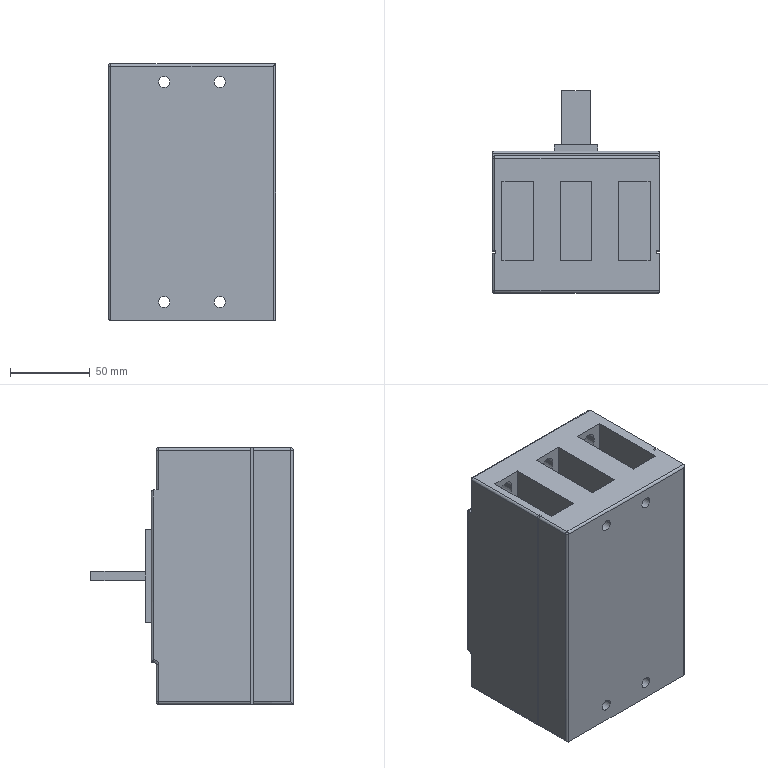Component | SolidWorks | NSX100F-3PMoldedCase-1 | 1 solid | 119 faces | volume 1318106 mm3 | plane 75 | cylinder 39 | sphere 3 | torus 2 | commonest cylinder face diameters 3 x19 10 x12 7 x8